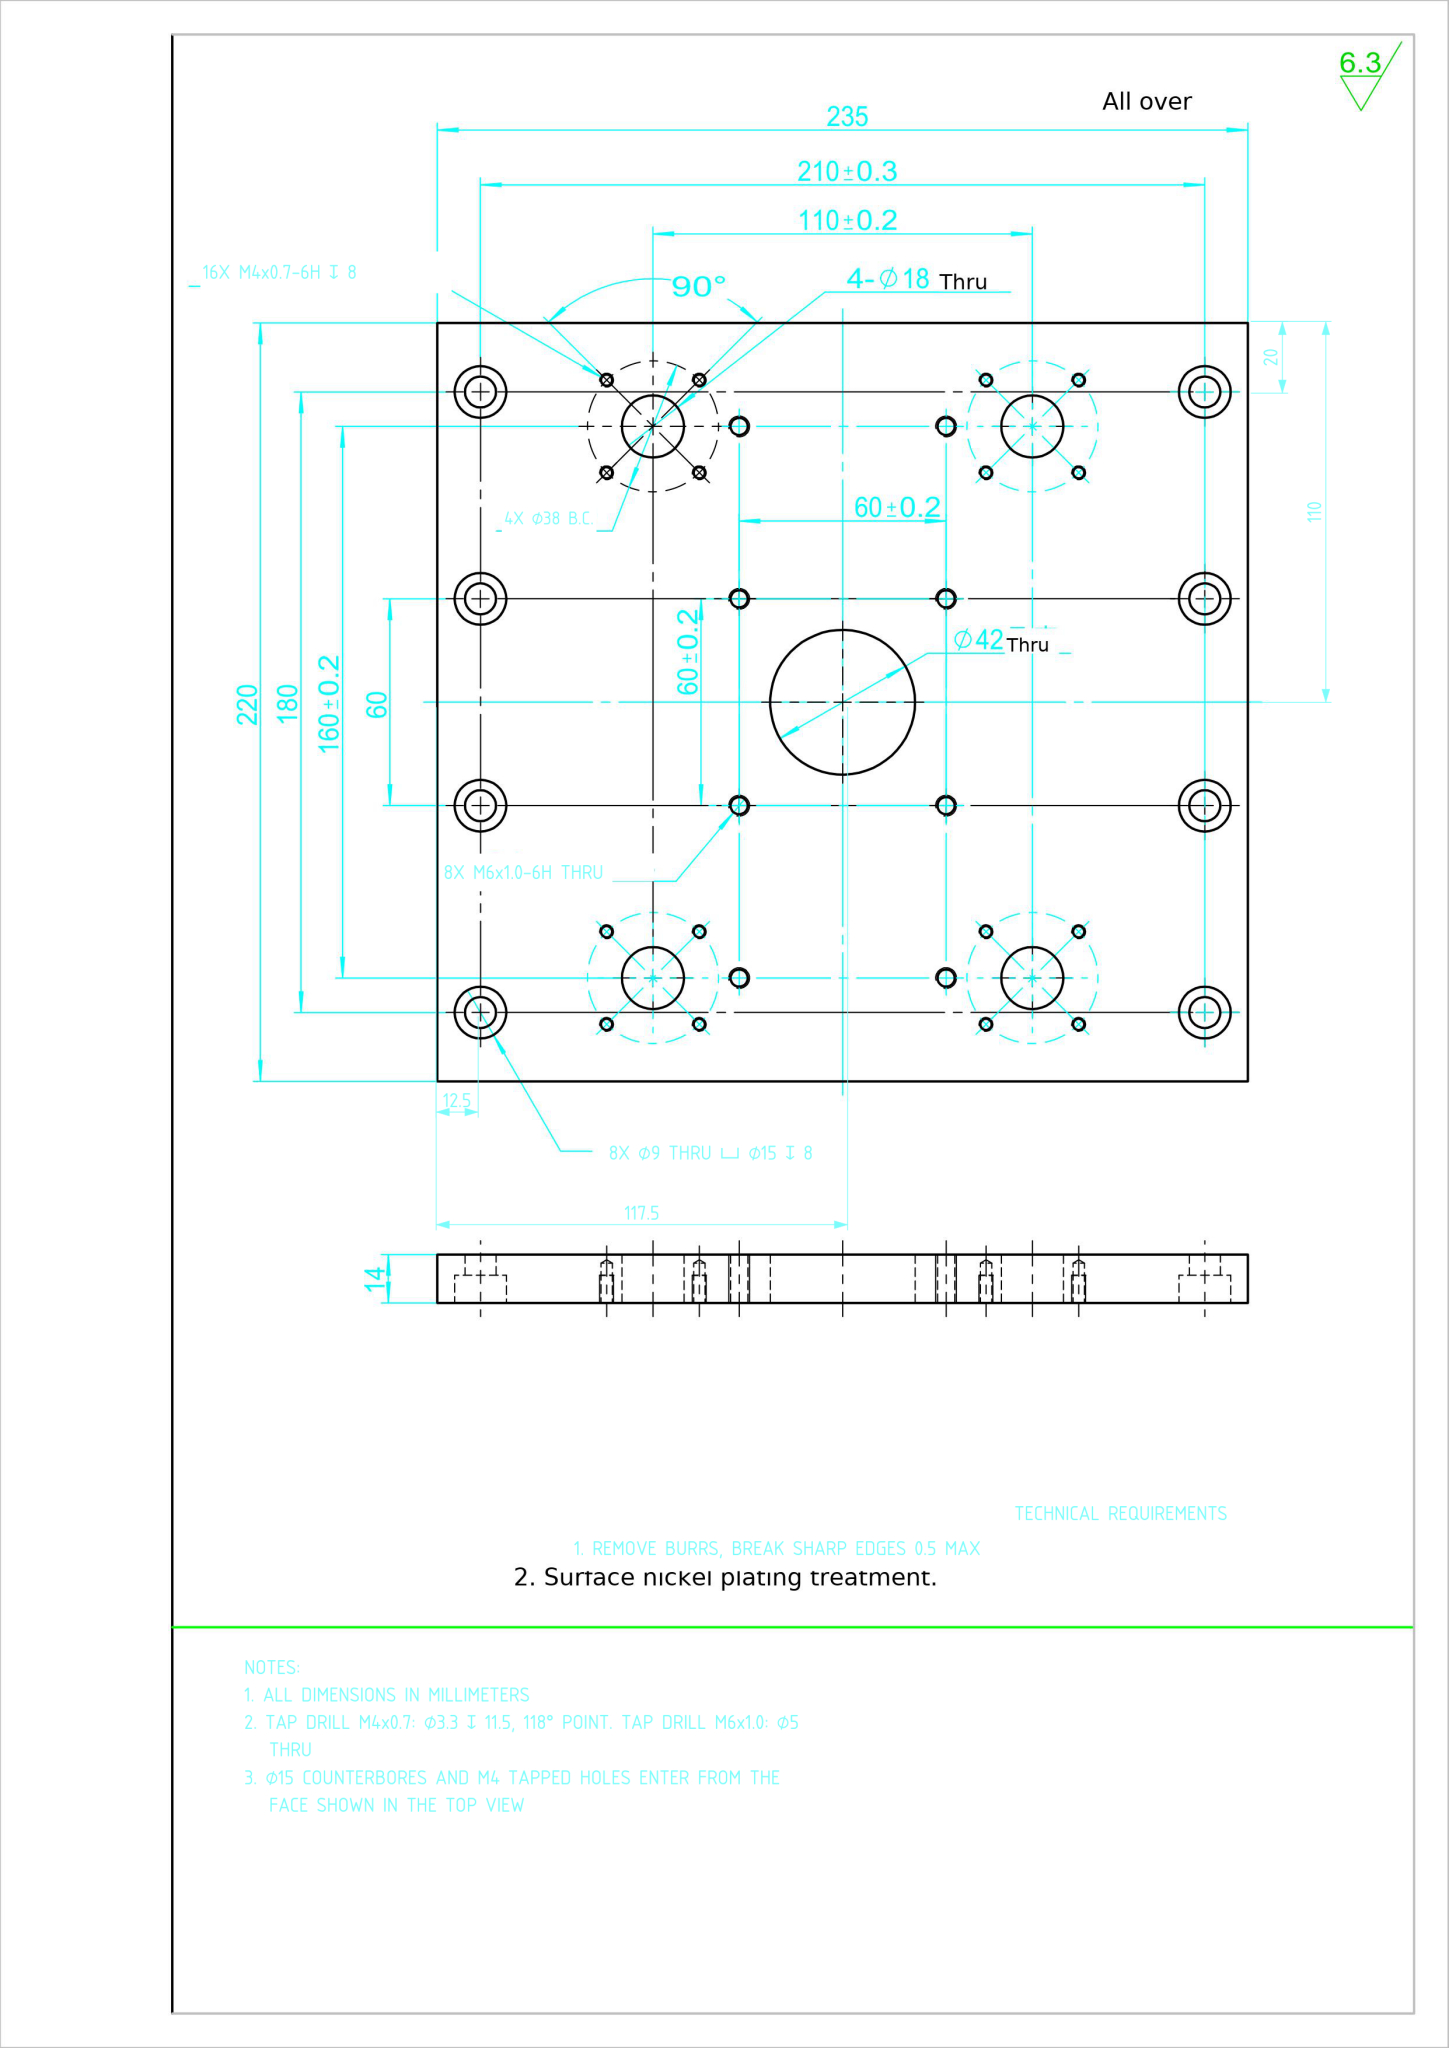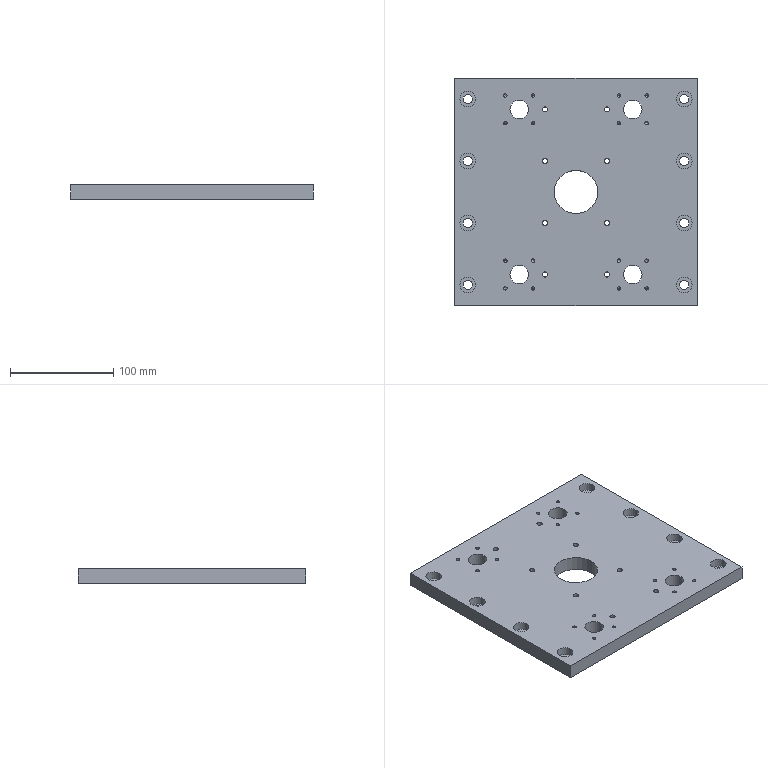Part | NX | mm | 1 solid | 136 faces | box 235 x 220 x 14 mm | volume 671972 mm3 | cylinder 90 | cone 32 | plane 14 | commonest cylinder face diameters 3.3 x32 15 x16 9 x16 5 x16 18 x8 42 x2